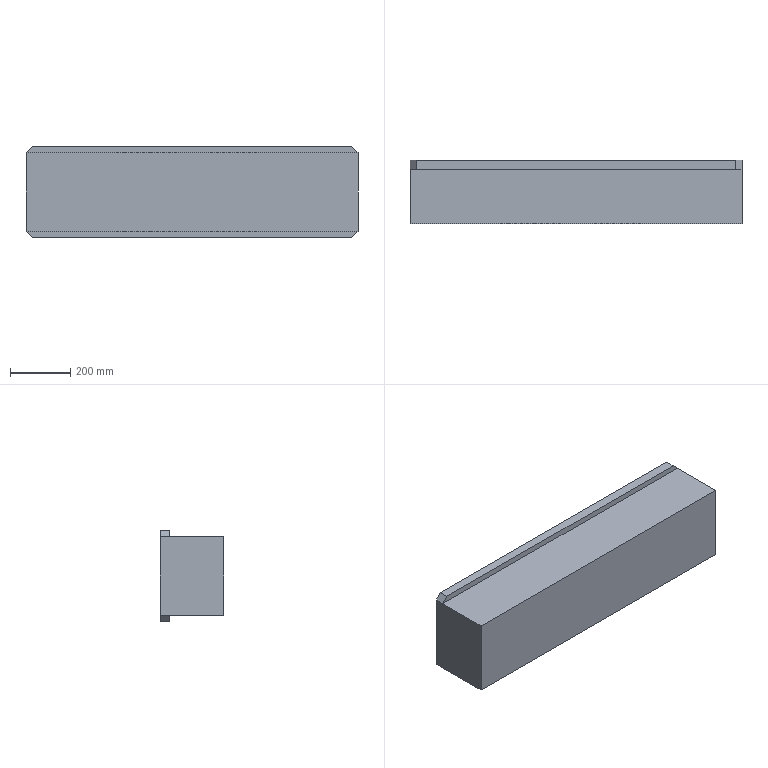Component | SolidWorks | -3[3]-1 | 1 solid | 26 faces | box 1100 x 210 x 300 mm | volume 61122548 mm3 | plane 18 | cylinder 8 | commonest cylinder face diameters 65 x4 27 x4
STEP:
#1=COLOUR_RGB('',0.7922,0.8196,0.9333);
#2=FILL_AREA_STYLE_COLOUR('',#1);
#3=FILL_AREA_STYLE('',(#2));
#4=SURFACE_STYLE_FILL_AREA(#3);
#5=SURFACE_SIDE_STYLE('',(#4));
#6=SURFACE_STYLE_USAGE(.BOTH.,#5);
#7=PRESENTATION_STYLE_ASSIGNMENT((#6));
#8=CARTESIAN_POINT('',(19.685,-89.764,47.736));
#9=VERTEX_POINT('',#8);
#10=CARTESIAN_POINT('',(19.685,-89.764,45.177));
#11=VERTEX_POINT('',#10);
#12=CARTESIAN_POINT('',(19.685,-89.764,46.457));
#13=DIRECTION('',(0.,-1.,0.));
#14=DIRECTION('',(0.,0.,1.));
#15=AXIS2_PLACEMENT_3D('',#12,#13,#14);
#16=CIRCLE('',#15,1.28);
#17=EDGE_CURVE('',#9,#11,#16,.T.);
#18=ORIENTED_EDGE('',*,*,#17,.T.);
#19=CARTESIAN_POINT('',(19.685,-88.583,45.177));
#20=VERTEX_POINT('',#19);
#21=CARTESIAN_POINT('',(19.685,-89.764,45.177));
#22=DIRECTION('',(0.,1.,0.));
#23=VECTOR('',#22,39.37);
#24=LINE('',#21,#23);
#25=EDGE_CURVE('',#11,#20,#24,.T.);
#26=ORIENTED_EDGE('',*,*,#25,.T.);
#27=CARTESIAN_POINT('',(19.685,-88.583,47.736));
#28=VERTEX_POINT('',#27);
#29=CARTESIAN_POINT('',(19.685,-88.583,46.457));
#30=DIRECTION('',(0.,-1.,0.));
#31=DIRECTION('',(0.,0.,1.));
#32=AXIS2_PLACEMENT_3D('',#29,#30,#31);
#33=CIRCLE('',#32,1.28);
#34=EDGE_CURVE('',#28,#20,#33,.T.);
#35=ORIENTED_EDGE('',*,*,#34,.F.);
#36=CARTESIAN_POINT('',(19.685,-89.764,47.736));
#37=DIRECTION('',(0.,1.,0.));
#38=VECTOR('',#37,39.37);
#39=LINE('',#36,#38);
#40=EDGE_CURVE('',#9,#28,#39,.T.);
#41=ORIENTED_EDGE('',*,*,#40,.F.);
#42=EDGE_LOOP('',(#18,#26,#35,#41));
#43=FACE_OUTER_BOUND('',#42,.T.);
#44=CARTESIAN_POINT('',(19.685,-89.764,46.457));
#45=DIRECTION('',(0.,1.,0.));
#46=DIRECTION('',(0.,0.,-1.));
#47=AXIS2_PLACEMENT_3D('',#44,#45,#46);
#48=CYLINDRICAL_SURFACE('',#47,1.28);
#49=ADVANCED_FACE('',(#43),#48,.F.);
#50=CARTESIAN_POINT('',(19.685,-89.764,43.839));
#51=VERTEX_POINT('',#50);
#52=CARTESIAN_POINT('',(19.685,-89.764,42.776));
#53=VERTEX_POINT('',#52);
#54=CARTESIAN_POINT('',(19.685,-89.764,43.307));
#55=DIRECTION('',(0.,-1.,0.));
#56=DIRECTION('',(0.,0.,1.));
#57=AXIS2_PLACEMENT_3D('',#54,#55,#56);
#58=CIRCLE('',#57,0.5315);
#59=EDGE_CURVE('',#51,#53,#58,.T.);
#60=ORIENTED_EDGE('',*,*,#59,.T.);
#61=CARTESIAN_POINT('',(19.685,-88.583,42.776));
#62=VERTEX_POINT('',#61);
#63=CARTESIAN_POINT('',(19.685,-89.764,42.776));
#64=DIRECTION('',(0.,1.,0.));
#65=VECTOR('',#64,39.37);
#66=LINE('',#63,#65);
#67=EDGE_CURVE('',#53,#62,#66,.T.);
#68=ORIENTED_EDGE('',*,*,#67,.T.);
#69=CARTESIAN_POINT('',(19.685,-88.583,43.839));
#70=VERTEX_POINT('',#69);
#71=CARTESIAN_POINT('',(19.685,-88.583,43.307));
#72=DIRECTION('',(0.,-1.,0.));
#73=DIRECTION('',(0.,0.,1.));
#74=AXIS2_PLACEMENT_3D('',#71,#72,#73);
#75=CIRCLE('',#74,0.5315);
#76=EDGE_CURVE('',#70,#62,#75,.T.);
#77=ORIENTED_EDGE('',*,*,#76,.F.);
#78=CARTESIAN_POINT('',(19.685,-89.764,43.839));
#79=DIRECTION('',(0.,1.,0.));
#80=VECTOR('',#79,39.37);
#81=LINE('',#78,#80);
#82=EDGE_CURVE('',#51,#70,#81,.T.);
#83=ORIENTED_EDGE('',*,*,#82,.F.);
#84=EDGE_LOOP('',(#60,#68,#77,#83));
#85=FACE_OUTER_BOUND('',#84,.T.);
#86=CARTESIAN_POINT('',(19.685,-89.764,43.307));
#87=DIRECTION('',(0.,1.,0.));
#88=DIRECTION('',(0.,0.,-1.));
#89=AXIS2_PLACEMENT_3D('',#86,#87,#88);
#90=CYLINDRICAL_SURFACE('',#89,0.5315);
#91=ADVANCED_FACE('',(#85),#90,.F.);
#92=CARTESIAN_POINT('',(-19.685,-89.764,43.839));
#93=VERTEX_POINT('',#92);
#94=CARTESIAN_POINT('',(-19.685,-89.764,42.776));
#95=VERTEX_POINT('',#94);
#96=CARTESIAN_POINT('',(-19.685,-89.764,43.307));
#97=DIRECTION('',(0.,-1.,0.));
#98=DIRECTION('',(0.,0.,-1.));
#99=AXIS2_PLACEMENT_3D('',#96,#97,#98);
#100=CIRCLE('',#99,0.5315);
#101=EDGE_CURVE('',#93,#95,#100,.T.);
#102=ORIENTED_EDGE('',*,*,#101,.T.);
#103=CARTESIAN_POINT('',(-19.685,-88.583,42.776));
#104=VERTEX_POINT('',#103);
#105=CARTESIAN_POINT('',(-19.685,-89.764,42.776));
#106=DIRECTION('',(0.,1.,0.));
#107=VECTOR('',#106,39.37);
#108=LINE('',#105,#107);
#109=EDGE_CURVE('',#95,#104,#108,.T.);
#110=ORIENTED_EDGE('',*,*,#109,.T.);
#111=CARTESIAN_POINT('',(-19.685,-88.583,43.839));
#112=VERTEX_POINT('',#111);
#113=CARTESIAN_POINT('',(-19.685,-88.583,43.307));
#114=DIRECTION('',(0.,-1.,0.));
#115=DIRECTION('',(0.,0.,-1.));
#116=AXIS2_PLACEMENT_3D('',#113,#114,#115);
#117=CIRCLE('',#116,0.5315);
#118=EDGE_CURVE('',#112,#104,#117,.T.);
#119=ORIENTED_EDGE('',*,*,#118,.F.);
#120=CARTESIAN_POINT('',(-19.685,-89.764,43.839));
#121=DIRECTION('',(0.,1.,0.));
#122=VECTOR('',#121,39.37);
#123=LINE('',#120,#122);
#124=EDGE_CURVE('',#93,#112,#123,.T.);
#125=ORIENTED_EDGE('',*,*,#124,.F.);
#126=EDGE_LOOP('',(#102,#110,#119,#125));
#127=FACE_OUTER_BOUND('',#126,.T.);
#128=CARTESIAN_POINT('',(-19.685,-89.764,43.307));
#129=DIRECTION('',(0.,1.,0.));
#130=DIRECTION('',(0.,0.,-1.));
#131=AXIS2_PLACEMENT_3D('',#128,#129,#130);
#132=CYLINDRICAL_SURFACE('',#131,0.5315);
#133=ADVANCED_FACE('',(#127),#132,.F.);
#134=CARTESIAN_POINT('',(-19.685,-89.764,47.736));
#135=VERTEX_POINT('',#134);
#136=CARTESIAN_POINT('',(-19.685,-89.764,45.177));
#137=VERTEX_POINT('',#136);
#138=CARTESIAN_POINT('',(-19.685,-89.764,46.457));
#139=DIRECTION('',(0.,-1.,0.));
#140=DIRECTION('',(0.,0.,-1.));
#141=AXIS2_PLACEMENT_3D('',#138,#139,#140);
#142=CIRCLE('',#141,1.28);
#143=EDGE_CURVE('',#135,#137,#142,.T.);
#144=ORIENTED_EDGE('',*,*,#143,.T.);
#145=CARTESIAN_POINT('',(-19.685,-88.583,45.177));
#146=VERTEX_POINT('',#145);
#147=CARTESIAN_POINT('',(-19.685,-89.764,45.177));
#148=DIRECTION('',(0.,1.,0.));
#149=VECTOR('',#148,39.37);
#150=LINE('',#147,#149);
#151=EDGE_CURVE('',#137,#146,#150,.T.);
#152=ORIENTED_EDGE('',*,*,#151,.T.);
#153=CARTESIAN_POINT('',(-19.685,-88.583,47.736));
#154=VERTEX_POINT('',#153);
#155=CARTESIAN_POINT('',(-19.685,-88.583,46.457));
#156=DIRECTION('',(0.,-1.,0.));
#157=DIRECTION('',(0.,0.,-1.));
#158=AXIS2_PLACEMENT_3D('',#155,#156,#157);
#159=CIRCLE('',#158,1.28);
#160=EDGE_CURVE('',#154,#146,#159,.T.);
#161=ORIENTED_EDGE('',*,*,#160,.F.);
#162=CARTESIAN_POINT('',(-19.685,-89.764,47.736));
#163=DIRECTION('',(0.,1.,0.));
#164=VECTOR('',#163,39.37);
#165=LINE('',#162,#164);
#166=EDGE_CURVE('',#135,#154,#165,.T.);
#167=ORIENTED_EDGE('',*,*,#166,.F.);
#168=EDGE_LOOP('',(#144,#152,#161,#167));
#169=FACE_OUTER_BOUND('',#168,.T.);
#170=CARTESIAN_POINT('',(-19.685,-89.764,46.457));
#171=DIRECTION('',(0.,1.,0.));
#172=DIRECTION('',(0.,0.,-1.));
#173=AXIS2_PLACEMENT_3D('',#170,#171,#172);
#174=CYLINDRICAL_SURFACE('',#173,1.28);
#175=ADVANCED_FACE('',(#169),#174,.F.);
#176=CARTESIAN_POINT('',(21.654,-89.764,50.394));
#177=VERTEX_POINT('',#176);
#178=CARTESIAN_POINT('',(-21.654,-89.764,50.394));
#179=VERTEX_POINT('',#178);
#180=CARTESIAN_POINT('',(-21.654,-89.764,50.394));
#181=DIRECTION('',(-1.,0.,0.));
#182=VECTOR('',#181,39.37);
#183=LINE('',#180,#182);
#184=EDGE_CURVE('',#177,#179,#183,.T.);
#185=ORIENTED_EDGE('',*,*,#184,.F.);
#186=CARTESIAN_POINT('',(20.866,-89.764,51.181));
#187=VERTEX_POINT('',#186);
#188=CARTESIAN_POINT('',(20.866,-89.764,51.181));
#189=DIRECTION('',(-0.7071,0.,0.7071));
#190=VECTOR('',#189,39.37);
#191=LINE('',#188,#190);
#192=EDGE_CURVE('',#177,#187,#191,.T.);
#193=ORIENTED_EDGE('',*,*,#192,.T.);
#194=CARTESIAN_POINT('',(-20.866,-89.764,51.181));
#195=VERTEX_POINT('',#194);
#196=CARTESIAN_POINT('',(-20.866,-89.764,51.181));
#197=DIRECTION('',(-1.,0.,-0.));
#198=VECTOR('',#197,39.37);
#199=LINE('',#196,#198);
#200=EDGE_CURVE('',#187,#195,#199,.T.);
#201=ORIENTED_EDGE('',*,*,#200,.T.);
#202=CARTESIAN_POINT('',(-21.654,-89.764,50.394));
#203=DIRECTION('',(-0.7071,0.,-0.7071));
#204=VECTOR('',#203,39.37);
#205=LINE('',#202,#204);
#206=EDGE_CURVE('',#195,#179,#205,.T.);
#207=ORIENTED_EDGE('',*,*,#206,.T.);
#208=EDGE_LOOP('',(#185,#193,#201,#207));
#209=FACE_OUTER_BOUND('',#208,.T.);
#210=CARTESIAN_POINT('',(0.,-89.764,72.047));
#211=DIRECTION('',(0.,1.,0.));
#212=DIRECTION('',(0.,0.,-1.));
#213=AXIS2_PLACEMENT_3D('',#210,#211,#212);
#214=PLANE('',#213);
#215=ADVANCED_FACE('',(#209),#214,.F.);
#216=CARTESIAN_POINT('',(-21.654,-89.764,40.157));
#217=VERTEX_POINT('',#216);
#218=CARTESIAN_POINT('',(21.654,-89.764,40.157));
#219=VERTEX_POINT('',#218);
#220=CARTESIAN_POINT('',(-21.654,-89.764,40.157));
#221=DIRECTION('',(1.,0.,0.));
#222=VECTOR('',#221,39.37);
#223=LINE('',#220,#222);
#224=EDGE_CURVE('',#217,#219,#223,.T.);
#225=ORIENTED_EDGE('',*,*,#224,.F.);
#226=CARTESIAN_POINT('',(-20.866,-89.764,39.37));
#227=VERTEX_POINT('',#226);
#228=CARTESIAN_POINT('',(-21.654,-89.764,40.157));
#229=DIRECTION('',(0.7071,0.,-0.7071));
#230=VECTOR('',#229,39.37);
#231=LINE('',#228,#230);
#232=EDGE_CURVE('',#217,#227,#231,.T.);
#233=ORIENTED_EDGE('',*,*,#232,.T.);
#234=CARTESIAN_POINT('',(20.866,-89.764,39.37));
#235=VERTEX_POINT('',#234);
#236=CARTESIAN_POINT('',(-20.866,-89.764,39.37));
#237=DIRECTION('',(1.,0.,0.));
#238=VECTOR('',#237,39.37);
#239=LINE('',#236,#238);
#240=EDGE_CURVE('',#227,#235,#239,.T.);
#241=ORIENTED_EDGE('',*,*,#240,.T.);
#242=CARTESIAN_POINT('',(21.654,-89.764,40.157));
#243=DIRECTION('',(0.7071,0.,0.7071));
#244=VECTOR('',#243,39.37);
#245=LINE('',#242,#244);
#246=EDGE_CURVE('',#235,#219,#245,.T.);
#247=ORIENTED_EDGE('',*,*,#246,.T.);
#248=EDGE_LOOP('',(#225,#233,#241,#247));
#249=FACE_OUTER_BOUND('',#248,.T.);
#250=CARTESIAN_POINT('',(0.,-89.764,72.047));
#251=DIRECTION('',(0.,1.,0.));
#252=DIRECTION('',(0.,0.,-1.));
#253=AXIS2_PLACEMENT_3D('',#250,#251,#252);
#254=PLANE('',#253);
#255=ADVANCED_FACE('',(#249),#254,.F.);
#256=ORIENTED_EDGE('',*,*,#76,.T.);
#257=CARTESIAN_POINT('',(19.685,-88.583,43.307));
#258=DIRECTION('',(0.,-1.,0.));
#259=DIRECTION('',(0.,0.,1.));
#260=AXIS2_PLACEMENT_3D('',#257,#258,#259);
#261=CIRCLE('',#260,0.5315);
#262=EDGE_CURVE('',#62,#70,#261,.T.);
#263=ORIENTED_EDGE('',*,*,#262,.T.);
#264=EDGE_LOOP('',(#256,#263));
#265=FACE_BOUND('',#264,.T.);
#266=ORIENTED_EDGE('',*,*,#160,.T.);
#267=CARTESIAN_POINT('',(-19.685,-88.583,46.457));
#268=DIRECTION('',(0.,-1.,0.));
#269=DIRECTION('',(0.,0.,-1.));
#270=AXIS2_PLACEMENT_3D('',#267,#268,#269);
#271=CIRCLE('',#270,1.28);
#272=EDGE_CURVE('',#146,#154,#271,.T.);
#273=ORIENTED_EDGE('',*,*,#272,.T.);
#274=EDGE_LOOP('',(#266,#273));
#275=FACE_BOUND('',#274,.T.);
#276=CARTESIAN_POINT('',(-20.866,-88.583,51.181));
#277=VERTEX_POINT('',#276);
#278=CARTESIAN_POINT('',(-21.654,-88.583,50.394));
#279=VERTEX_POINT('',#278);
#280=CARTESIAN_POINT('',(-21.654,-88.583,50.394));
#281=DIRECTION('',(-0.7071,0.,-0.7071));
#282=VECTOR('',#281,39.37);
#283=LINE('',#280,#282);
#284=EDGE_CURVE('',#277,#279,#283,.T.);
#285=ORIENTED_EDGE('',*,*,#284,.F.);
#286=CARTESIAN_POINT('',(20.866,-88.583,51.181));
#287=VERTEX_POINT('',#286);
#288=CARTESIAN_POINT('',(-20.866,-88.583,51.181));
#289=DIRECTION('',(-1.,0.,-0.));
#290=VECTOR('',#289,39.37);
#291=LINE('',#288,#290);
#292=EDGE_CURVE('',#287,#277,#291,.T.);
#293=ORIENTED_EDGE('',*,*,#292,.F.);
#294=CARTESIAN_POINT('',(21.654,-88.583,50.394));
#295=VERTEX_POINT('',#294);
#296=CARTESIAN_POINT('',(20.866,-88.583,51.181));
#297=DIRECTION('',(-0.7071,0.,0.7071));
#298=VECTOR('',#297,39.37);
#299=LINE('',#296,#298);
#300=EDGE_CURVE('',#295,#287,#299,.T.);
#301=ORIENTED_EDGE('',*,*,#300,.F.);
#302=CARTESIAN_POINT('',(21.654,-88.583,40.157));
#303=VERTEX_POINT('',#302);
#304=CARTESIAN_POINT('',(21.654,-88.583,50.394));
#305=DIRECTION('',(0.,0.,1.));
#306=VECTOR('',#305,39.37);
#307=LINE('',#304,#306);
#308=EDGE_CURVE('',#303,#295,#307,.T.);
#309=ORIENTED_EDGE('',*,*,#308,.F.);
#310=CARTESIAN_POINT('',(20.866,-88.583,39.37));
#311=VERTEX_POINT('',#310);
#312=CARTESIAN_POINT('',(21.654,-88.583,40.157));
#313=DIRECTION('',(0.7071,0.,0.7071));
#314=VECTOR('',#313,39.37);
#315=LINE('',#312,#314);
#316=EDGE_CURVE('',#311,#303,#315,.T.);
#317=ORIENTED_EDGE('',*,*,#316,.F.);
#318=CARTESIAN_POINT('',(-20.866,-88.583,39.37));
#319=VERTEX_POINT('',#318);
#320=CARTESIAN_POINT('',(-20.866,-88.583,39.37));
#321=DIRECTION('',(1.,0.,0.));
#322=VECTOR('',#321,39.37);
#323=LINE('',#320,#322);
#324=EDGE_CURVE('',#319,#311,#323,.T.);
#325=ORIENTED_EDGE('',*,*,#324,.F.);
#326=CARTESIAN_POINT('',(-21.654,-88.583,40.157));
#327=VERTEX_POINT('',#326);
#328=CARTESIAN_POINT('',(-21.654,-88.583,40.157));
#329=DIRECTION('',(0.7071,0.,-0.7071));
#330=VECTOR('',#329,39.37);
#331=LINE('',#328,#330);
#332=EDGE_CURVE('',#327,#319,#331,.T.);
#333=ORIENTED_EDGE('',*,*,#332,.F.);
#334=CARTESIAN_POINT('',(-21.654,-88.583,50.394));
#335=DIRECTION('',(0.,0.,-1.));
#336=VECTOR('',#335,39.37);
#337=LINE('',#334,#336);
#338=EDGE_CURVE('',#279,#327,#337,.T.);
#339=ORIENTED_EDGE('',*,*,#338,.F.);
#340=EDGE_LOOP('',(#285,#293,#301,#309,#317,#325,#333,#339));
#341=FACE_OUTER_BOUND('',#340,.T.);
#342=ORIENTED_EDGE('',*,*,#118,.T.);
#343=CARTESIAN_POINT('',(-19.685,-88.583,43.307));
#344=DIRECTION('',(0.,-1.,0.));
#345=DIRECTION('',(0.,0.,-1.));
#346=AXIS2_PLACEMENT_3D('',#343,#344,#345);
#347=CIRCLE('',#346,0.5315);
#348=EDGE_CURVE('',#104,#112,#347,.T.);
#349=ORIENTED_EDGE('',*,*,#348,.T.);
#350=EDGE_LOOP('',(#342,#349));
#351=FACE_BOUND('',#350,.T.);
#352=ORIENTED_EDGE('',*,*,#34,.T.);
#353=CARTESIAN_POINT('',(19.685,-88.583,46.457));
#354=DIRECTION('',(0.,-1.,0.));
#355=DIRECTION('',(0.,0.,1.));
#356=AXIS2_PLACEMENT_3D('',#353,#354,#355);
#357=CIRCLE('',#356,1.28);
#358=EDGE_CURVE('',#20,#28,#357,.T.);
#359=ORIENTED_EDGE('',*,*,#358,.T.);
#360=EDGE_LOOP('',(#352,#359));
#361=FACE_BOUND('',#360,.T.);
#362=CARTESIAN_POINT('',(0.,-88.583,72.047));
#363=DIRECTION('',(0.,1.,0.));
#364=DIRECTION('',(0.,0.,-1.));
#365=AXIS2_PLACEMENT_3D('',#362,#363,#364);
#366=PLANE('',#365);
#367=ADVANCED_FACE('',(#265,#275,#341,#351,#361),#366,.T.);
#368=ORIENTED_EDGE('',*,*,#284,.T.);
#369=CARTESIAN_POINT('',(-21.654,-89.764,50.394));
#370=DIRECTION('',(0.,1.,0.));
#371=VECTOR('',#370,39.37);
#372=LINE('',#369,#371);
#373=EDGE_CURVE('',#179,#279,#372,.T.);
#374=ORIENTED_EDGE('',*,*,#373,.F.);
#375=ORIENTED_EDGE('',*,*,#206,.F.);
#376=CARTESIAN_POINT('',(-20.866,-89.764,51.181));
#377=DIRECTION('',(0.,1.,0.));
#378=VECTOR('',#377,39.37);
#379=LINE('',#376,#378);
#380=EDGE_CURVE('',#195,#277,#379,.T.);
#381=ORIENTED_EDGE('',*,*,#380,.T.);
#382=EDGE_LOOP('',(#368,#374,#375,#381));
#383=FACE_OUTER_BOUND('',#382,.T.);
#384=CARTESIAN_POINT('',(-21.654,-89.764,50.394));
#385=DIRECTION('',(0.7071,0.,-0.7071));
#386=DIRECTION('',(0.7071,0.,0.7071));
#387=AXIS2_PLACEMENT_3D('',#384,#385,#386);
#388=PLANE('',#387);
#389=ADVANCED_FACE('',(#383),#388,.F.);
#390=ORIENTED_EDGE('',*,*,#338,.T.);
#391=CARTESIAN_POINT('',(-21.654,-89.764,40.157));
#392=DIRECTION('',(0.,1.,0.));
#393=VECTOR('',#392,39.37);
#394=LINE('',#391,#393);
#395=EDGE_CURVE('',#217,#327,#394,.T.);
#396=ORIENTED_EDGE('',*,*,#395,.F.);
#397=CARTESIAN_POINT('',(-21.654,-96.85,40.157));
#398=VERTEX_POINT('',#397);
#399=CARTESIAN_POINT('',(-21.654,-96.85,40.157));
#400=DIRECTION('',(0.,1.,0.));
#401=VECTOR('',#400,39.37);
#402=LINE('',#399,#401);
#403=EDGE_CURVE('',#398,#217,#402,.T.);
#404=ORIENTED_EDGE('',*,*,#403,.F.);
#405=CARTESIAN_POINT('',(-21.654,-96.85,50.394));
#406=VERTEX_POINT('',#405);
#407=CARTESIAN_POINT('',(-21.654,-96.85,50.394));
#408=DIRECTION('',(0.,0.,-1.));
#409=VECTOR('',#408,39.37);
#410=LINE('',#407,#409);
#411=EDGE_CURVE('',#406,#398,#410,.T.);
#412=ORIENTED_EDGE('',*,*,#411,.F.);
#413=CARTESIAN_POINT('',(-21.654,-96.85,50.394));
#414=DIRECTION('',(0.,1.,0.));
#415=VECTOR('',#414,39.37);
#416=LINE('',#413,#415);
#417=EDGE_CURVE('',#406,#179,#416,.T.);
#418=ORIENTED_EDGE('',*,*,#417,.T.);
#419=ORIENTED_EDGE('',*,*,#373,.T.);
#420=EDGE_LOOP('',(#390,#396,#404,#412,#418,#419));
#421=FACE_OUTER_BOUND('',#420,.T.);
#422=CARTESIAN_POINT('',(-21.654,-89.764,50.394));
#423=DIRECTION('',(1.,0.,0.));
#424=DIRECTION('',(-0.,0.,1.));
#425=AXIS2_PLACEMENT_3D('',#422,#423,#424);
#426=PLANE('',#425);
#427=ADVANCED_FACE('',(#421),#426,.F.);
#428=ORIENTED_EDGE('',*,*,#332,.T.);
#429=CARTESIAN_POINT('',(-20.866,-89.764,39.37));
#430=DIRECTION('',(0.,1.,0.));
#431=VECTOR('',#430,39.37);
#432=LINE('',#429,#431);
#433=EDGE_CURVE('',#227,#319,#432,.T.);
#434=ORIENTED_EDGE('',*,*,#433,.F.);
#435=ORIENTED_EDGE('',*,*,#232,.F.);
#436=ORIENTED_EDGE('',*,*,#395,.T.);
#437=EDGE_LOOP('',(#428,#434,#435,#436));
#438=FACE_OUTER_BOUND('',#437,.T.);
#439=CARTESIAN_POINT('',(-21.654,-89.764,40.157));
#440=DIRECTION('',(0.7071,0.,0.7071));
#441=DIRECTION('',(-0.7071,0.,0.7071));
#442=AXIS2_PLACEMENT_3D('',#439,#440,#441);
#443=PLANE('',#442);
#444=ADVANCED_FACE('',(#438),#443,.F.);
#445=ORIENTED_EDGE('',*,*,#324,.T.);
#446=CARTESIAN_POINT('',(20.866,-89.764,39.37));
#447=DIRECTION('',(0.,1.,0.));
#448=VECTOR('',#447,39.37);
#449=LINE('',#446,#448);
#450=EDGE_CURVE('',#235,#311,#449,.T.);
#451=ORIENTED_EDGE('',*,*,#450,.F.);
#452=ORIENTED_EDGE('',*,*,#240,.F.);
#453=ORIENTED_EDGE('',*,*,#433,.T.);
#454=EDGE_LOOP('',(#445,#451,#452,#453));
#455=FACE_OUTER_BOUND('',#454,.T.);
#456=CARTESIAN_POINT('',(-20.866,-89.764,39.37));
#457=DIRECTION('',(-0.,0.,1.));
#458=DIRECTION('',(-1.,0.,-0.));
#459=AXIS2_PLACEMENT_3D('',#456,#457,#458);
#460=PLANE('',#459);
#461=ADVANCED_FACE('',(#455),#460,.F.);
#462=ORIENTED_EDGE('',*,*,#316,.T.);
#463=CARTESIAN_POINT('',(21.654,-89.764,40.157));
#464=DIRECTION('',(0.,1.,0.));
#465=VECTOR('',#464,39.37);
#466=LINE('',#463,#465);
#467=EDGE_CURVE('',#219,#303,#466,.T.);
#468=ORIENTED_EDGE('',*,*,#467,.F.);
#469=ORIENTED_EDGE('',*,*,#246,.F.);
#470=ORIENTED_EDGE('',*,*,#450,.T.);
#471=EDGE_LOOP('',(#462,#468,#469,#470));
#472=FACE_OUTER_BOUND('',#471,.T.);
#473=CARTESIAN_POINT('',(21.654,-89.764,40.157));
#474=DIRECTION('',(-0.7071,0.,0.7071));
#475=DIRECTION('',(-0.7071,0.,-0.7071));
#476=AXIS2_PLACEMENT_3D('',#473,#474,#475);
#477=PLANE('',#476);
#478=ADVANCED_FACE('',(#472),#477,.F.);
#479=ORIENTED_EDGE('',*,*,#308,.T.);
#480=CARTESIAN_POINT('',(21.654,-89.764,50.394));
#481=DIRECTION('',(0.,1.,0.));
#482=VECTOR('',#481,39.37);
#483=LINE('',#480,#482);
#484=EDGE_CURVE('',#177,#295,#483,.T.);
#485=ORIENTED_EDGE('',*,*,#484,.F.);
#486=CARTESIAN_POINT('',(21.654,-96.85,50.394));
#487=VERTEX_POINT('',#486);
#488=CARTESIAN_POINT('',(21.654,-96.85,50.394));
#489=DIRECTION('',(0.,1.,0.));
#490=VECTOR('',#489,39.37);
#491=LINE('',#488,#490);
#492=EDGE_CURVE('',#487,#177,#491,.T.);
#493=ORIENTED_EDGE('',*,*,#492,.F.);
#494=CARTESIAN_POINT('',(21.654,-96.85,40.157));
#495=VERTEX_POINT('',#494);
#496=CARTESIAN_POINT('',(21.654,-96.85,50.394));
#497=DIRECTION('',(0.,0.,1.));
#498=VECTOR('',#497,39.37);
#499=LINE('',#496,#498);
#500=EDGE_CURVE('',#495,#487,#499,.T.);
#501=ORIENTED_EDGE('',*,*,#500,.F.);
#502=CARTESIAN_POINT('',(21.654,-96.85,40.157));
#503=DIRECTION('',(0.,1.,0.));
#504=VECTOR('',#503,39.37);
#505=LINE('',#502,#504);
#506=EDGE_CURVE('',#495,#219,#505,.T.);
#507=ORIENTED_EDGE('',*,*,#506,.T.);
#508=ORIENTED_EDGE('',*,*,#467,.T.);
#509=EDGE_LOOP('',(#479,#485,#493,#501,#507,#508));
#510=FACE_OUTER_BOUND('',#509,.T.);
#511=CARTESIAN_POINT('',(21.654,-89.764,50.394));
#512=DIRECTION('',(-1.,0.,0.));
#513=DIRECTION('',(-0.,0.,-1.));
#514=AXIS2_PLACEMENT_3D('',#511,#512,#513);
#515=PLANE('',#514);
#516=ADVANCED_FACE('',(#510),#515,.F.);
#517=ORIENTED_EDGE('',*,*,#300,.T.);
#518=CARTESIAN_POINT('',(20.866,-89.764,51.181));
#519=DIRECTION('',(0.,1.,0.));
#520=VECTOR('',#519,39.37);
#521=LINE('',#518,#520);
#522=EDGE_CURVE('',#187,#287,#521,.T.);
#523=ORIENTED_EDGE('',*,*,#522,.F.);
#524=ORIENTED_EDGE('',*,*,#192,.F.);
#525=ORIENTED_EDGE('',*,*,#484,.T.);
#526=EDGE_LOOP('',(#517,#523,#524,#525));
#527=FACE_OUTER_BOUND('',#526,.T.);
#528=CARTESIAN_POINT('',(20.866,-89.764,51.181));
#529=DIRECTION('',(-0.7071,0.,-0.7071));
#530=DIRECTION('',(0.7071,0.,-0.7071));
#531=AXIS2_PLACEMENT_3D('',#528,#529,#530);
#532=PLANE('',#531);
#533=ADVANCED_FACE('',(#527),#532,.F.);
#534=ORIENTED_EDGE('',*,*,#292,.T.);
#535=ORIENTED_EDGE('',*,*,#380,.F.);
#536=ORIENTED_EDGE('',*,*,#200,.F.);
#537=ORIENTED_EDGE('',*,*,#522,.T.);
#538=EDGE_LOOP('',(#534,#535,#536,#537));
#539=FACE_OUTER_BOUND('',#538,.T.);
#540=CARTESIAN_POINT('',(-20.866,-89.764,51.181));
#541=DIRECTION('',(0.,0.,-1.));
#542=DIRECTION('',(1.,0.,0.));
#543=AXIS2_PLACEMENT_3D('',#540,#541,#542);
#544=PLANE('',#543);
#545=ADVANCED_FACE('',(#539),#544,.F.);
#546=ORIENTED_EDGE('',*,*,#151,.F.);
#547=CARTESIAN_POINT('',(-19.685,-89.764,46.457));
#548=DIRECTION('',(0.,-1.,0.));
#549=DIRECTION('',(0.,0.,-1.));
#550=AXIS2_PLACEMENT_3D('',#547,#548,#549);
#551=CIRCLE('',#550,1.28);
#552=EDGE_CURVE('',#137,#135,#551,.T.);
#553=ORIENTED_EDGE('',*,*,#552,.T.);
#554=ORIENTED_EDGE('',*,*,#166,.T.);
#555=ORIENTED_EDGE('',*,*,#272,.F.);
#556=EDGE_LOOP('',(#546,#553,#554,#555));
#557=FACE_OUTER_BOUND('',#556,.T.);
#558=CARTESIAN_POINT('',(-19.685,-89.764,46.457));
#559=DIRECTION('',(0.,1.,0.));
#560=DIRECTION('',(0.,0.,-1.));
#561=AXIS2_PLACEMENT_3D('',#558,#559,#560);
#562=CYLINDRICAL_SURFACE('',#561,1.28);
#563=ADVANCED_FACE('',(#557),#562,.F.);
#564=ORIENTED_EDGE('',*,*,#109,.F.);
#565=CARTESIAN_POINT('',(-19.685,-89.764,43.307));
#566=DIRECTION('',(0.,-1.,0.));
#567=DIRECTION('',(0.,0.,-1.));
#568=AXIS2_PLACEMENT_3D('',#565,#566,#567);
#569=CIRCLE('',#568,0.5315);
#570=EDGE_CURVE('',#95,#93,#569,.T.);
#571=ORIENTED_EDGE('',*,*,#570,.T.);
#572=ORIENTED_EDGE('',*,*,#124,.T.);
#573=ORIENTED_EDGE('',*,*,#348,.F.);
#574=EDGE_LOOP('',(#564,#571,#572,#573));
#575=FACE_OUTER_BOUND('',#574,.T.);
#576=CARTESIAN_POINT('',(-19.685,-89.764,43.307));
#577=DIRECTION('',(0.,1.,0.));
#578=DIRECTION('',(0.,0.,-1.));
#579=AXIS2_PLACEMENT_3D('',#576,#577,#578);
#580=CYLINDRICAL_SURFACE('',#579,0.5315);
#581=ADVANCED_FACE('',(#575),#580,.F.);
#582=ORIENTED_EDGE('',*,*,#67,.F.);
#583=CARTESIAN_POINT('',(19.685,-89.764,43.307));
#584=DIRECTION('',(0.,-1.,0.));
#585=DIRECTION('',(0.,0.,1.));
#586=AXIS2_PLACEMENT_3D('',#583,#584,#585);
#587=CIRCLE('',#586,0.5315);
#588=EDGE_CURVE('',#53,#51,#587,.T.);
#589=ORIENTED_EDGE('',*,*,#588,.T.);
#590=ORIENTED_EDGE('',*,*,#82,.T.);
#591=ORIENTED_EDGE('',*,*,#262,.F.);
#592=EDGE_LOOP('',(#582,#589,#590,#591));
#593=FACE_OUTER_BOUND('',#592,.T.);
#594=CARTESIAN_POINT('',(19.685,-89.764,43.307));
#595=DIRECTION('',(0.,1.,0.));
#596=DIRECTION('',(0.,0.,-1.));
#597=AXIS2_PLACEMENT_3D('',#594,#595,#596);
#598=CYLINDRICAL_SURFACE('',#597,0.5315);
#599=ADVANCED_FACE('',(#593),#598,.F.);
#600=ORIENTED_EDGE('',*,*,#25,.F.);
#601=CARTESIAN_POINT('',(19.685,-89.764,46.457));
#602=DIRECTION('',(0.,-1.,0.));
#603=DIRECTION('',(0.,0.,1.));
#604=AXIS2_PLACEMENT_3D('',#601,#602,#603);
#605=CIRCLE('',#604,1.28);
#606=EDGE_CURVE('',#11,#9,#605,.T.);
#607=ORIENTED_EDGE('',*,*,#606,.T.);
#608=ORIENTED_EDGE('',*,*,#40,.T.);
#609=ORIENTED_EDGE('',*,*,#358,.F.);
#610=EDGE_LOOP('',(#600,#607,#608,#609));
#611=FACE_OUTER_BOUND('',#610,.T.);
#612=CARTESIAN_POINT('',(19.685,-89.764,46.457));
#613=DIRECTION('',(0.,1.,0.));
#614=DIRECTION('',(0.,0.,-1.));
#615=AXIS2_PLACEMENT_3D('',#612,#613,#614);
#616=CYLINDRICAL_SURFACE('',#615,1.28);
#617=ADVANCED_FACE('',(#611),#616,.F.);
#618=ORIENTED_EDGE('',*,*,#411,.T.);
#619=CARTESIAN_POINT('',(-21.654,-96.85,40.157));
#620=DIRECTION('',(1.,0.,0.));
#621=VECTOR('',#620,39.37);
#622=LINE('',#619,#621);
#623=EDGE_CURVE('',#398,#495,#622,.T.);
#624=ORIENTED_EDGE('',*,*,#623,.T.);
#625=ORIENTED_EDGE('',*,*,#500,.T.);
#626=CARTESIAN_POINT('',(-21.654,-96.85,50.394));
#627=DIRECTION('',(-1.,0.,0.));
#628=VECTOR('',#627,39.37);
#629=LINE('',#626,#628);
#630=EDGE_CURVE('',#487,#406,#629,.T.);
#631=ORIENTED_EDGE('',*,*,#630,.T.);
#632=EDGE_LOOP('',(#618,#624,#625,#631));
#633=FACE_OUTER_BOUND('',#632,.T.);
#634=CARTESIAN_POINT('',(0.,-96.85,0.));
#635=DIRECTION('',(0.,-1.,0.));
#636=DIRECTION('',(0.,0.,1.));
#637=AXIS2_PLACEMENT_3D('',#634,#635,#636);
#638=PLANE('',#637);
#639=ADVANCED_FACE('',(#633),#638,.T.);
#640=ORIENTED_EDGE('',*,*,#184,.T.);
#641=ORIENTED_EDGE('',*,*,#417,.F.);
#642=ORIENTED_EDGE('',*,*,#630,.F.);
#643=ORIENTED_EDGE('',*,*,#492,.T.);
#644=EDGE_LOOP('',(#640,#641,#642,#643));
#645=FACE_OUTER_BOUND('',#644,.T.);
#646=CARTESIAN_POINT('',(-21.654,-96.85,50.394));
#647=DIRECTION('',(0.,0.,-1.));
#648=DIRECTION('',(1.,0.,0.));
#649=AXIS2_PLACEMENT_3D('',#646,#647,#648);
#650=PLANE('',#649);
#651=ADVANCED_FACE('',(#645),#650,.F.);
#652=ORIENTED_EDGE('',*,*,#224,.T.);
#653=ORIENTED_EDGE('',*,*,#506,.F.);
#654=ORIENTED_EDGE('',*,*,#623,.F.);
#655=ORIENTED_EDGE('',*,*,#403,.T.);
#656=EDGE_LOOP('',(#652,#653,#654,#655));
#657=FACE_OUTER_BOUND('',#656,.T.);
#658=CARTESIAN_POINT('',(-21.654,-96.85,40.157));
#659=DIRECTION('',(0.,0.,1.));
#660=DIRECTION('',(-1.,0.,0.));
#661=AXIS2_PLACEMENT_3D('',#658,#659,#660);
#662=PLANE('',#661);
#663=ADVANCED_FACE('',(#657),#662,.F.);
#664=ORIENTED_EDGE('',*,*,#17,.F.);
#665=ORIENTED_EDGE('',*,*,#606,.F.);
#666=EDGE_LOOP('',(#664,#665));
#667=FACE_OUTER_BOUND('',#666,.T.);
#668=CARTESIAN_POINT('',(0.,-89.764,0.));
#669=DIRECTION('',(0.,-1.,0.));
#670=DIRECTION('',(0.,0.,1.));
#671=AXIS2_PLACEMENT_3D('',#668,#669,#670);
#672=PLANE('',#671);
#673=ADVANCED_FACE('',(#667),#672,.F.);
#674=ORIENTED_EDGE('',*,*,#101,.F.);
#675=ORIENTED_EDGE('',*,*,#570,.F.);
#676=EDGE_LOOP('',(#674,#675));
#677=FACE_OUTER_BOUND('',#676,.T.);
#678=CARTESIAN_POINT('',(0.,-89.764,0.));
#679=DIRECTION('',(0.,-1.,0.));
#680=DIRECTION('',(0.,0.,1.));
#681=AXIS2_PLACEMENT_3D('',#678,#679,#680);
#682=PLANE('',#681);
#683=ADVANCED_FACE('',(#677),#682,.F.);
#684=ORIENTED_EDGE('',*,*,#143,.F.);
#685=ORIENTED_EDGE('',*,*,#552,.F.);
#686=EDGE_LOOP('',(#684,#685));
#687=FACE_OUTER_BOUND('',#686,.T.);
#688=CARTESIAN_POINT('',(0.,-89.764,0.));
#689=DIRECTION('',(0.,-1.,0.));
#690=DIRECTION('',(0.,0.,1.));
#691=AXIS2_PLACEMENT_3D('',#688,#689,#690);
#692=PLANE('',#691);
#693=ADVANCED_FACE('',(#687),#692,.F.);
#694=ORIENTED_EDGE('',*,*,#59,.F.);
#695=ORIENTED_EDGE('',*,*,#588,.F.);
#696=EDGE_LOOP('',(#694,#695));
#697=FACE_OUTER_BOUND('',#696,.T.);
#698=CARTESIAN_POINT('',(0.,-89.764,0.));
#699=DIRECTION('',(0.,-1.,0.));
#700=DIRECTION('',(0.,0.,1.));
#701=AXIS2_PLACEMENT_3D('',#698,#699,#700);
#702=PLANE('',#701);
#703=ADVANCED_FACE('',(#697),#702,.F.);
#704=CLOSED_SHELL('',(#49,#91,#133,#175,#215,#255,#367,#389,#427,#444,#461,#478,#516,#533,#545,#563,#581,#599,#617,#639,#651,#663,#673,#683,#693,#703));
#705=MANIFOLD_SOLID_BREP('',#704);
#706=STYLED_ITEM('',(#7),#705);
#707=(LENGTH_UNIT()NAMED_UNIT(*)SI_UNIT($,.METRE.));
#708=LENGTH_MEASURE_WITH_UNIT(LENGTH_MEASURE(0.0254),#707);
#709=DIMENSIONAL_EXPONENTS(1.,0.,0.,0.,0.,0.,0.);
#710=(CONVERSION_BASED_UNIT('',#708)LENGTH_UNIT()NAMED_UNIT(#709));
#711=UNCERTAINTY_MEASURE_WITH_UNIT(LENGTH_MEASURE(0.00001),#710,'','');
#712=(NAMED_UNIT(*)PLANE_ANGLE_UNIT()SI_UNIT($,.RADIAN.));
#713=(NAMED_UNIT(*)SI_UNIT($,.STERADIAN.)SOLID_ANGLE_UNIT());
#714=(GEOMETRIC_REPRESENTATION_CONTEXT(3)GLOBAL_UNCERTAINTY_ASSIGNED_CONTEXT((#711))GLOBAL_UNIT_ASSIGNED_CONTEXT((#710,#712,#713))REPRESENTATION_CONTEXT('',''));
#715=MECHANICAL_DESIGN_GEOMETRIC_PRESENTATION_REPRESENTATION('',(#706),#714);
#716=PRESENTATION_LAYER_ASSIGNMENT('','',(#706));
#717=CARTESIAN_POINT('',(0.,0.,0.));
#718=DIRECTION('',(0.,0.,1.));
#719=DIRECTION('',(1.,0.,0.));
#720=AXIS2_PLACEMENT_3D('',#717,#718,#719);
#721=(LENGTH_UNIT()NAMED_UNIT(*)SI_UNIT($,.METRE.));
#722=LENGTH_MEASURE_WITH_UNIT(LENGTH_MEASURE(0.0254),#721);
#723=DIMENSIONAL_EXPONENTS(1.,0.,0.,0.,0.,0.,0.);
#724=(CONVERSION_BASED_UNIT('',#722)LENGTH_UNIT()NAMED_UNIT(#723));
#725=UNCERTAINTY_MEASURE_WITH_UNIT(LENGTH_MEASURE(0.00001),#724,'','');
#726=(NAMED_UNIT(*)PLANE_ANGLE_UNIT()SI_UNIT($,.RADIAN.));
#727=(NAMED_UNIT(*)SI_UNIT($,.STERADIAN.)SOLID_ANGLE_UNIT());
#728=(GEOMETRIC_REPRESENTATION_CONTEXT(3)GLOBAL_UNCERTAINTY_ASSIGNED_CONTEXT((#725))GLOBAL_UNIT_ASSIGNED_CONTEXT((#724,#726,#727))REPRESENTATION_CONTEXT('',''));
#729=ADVANCED_BREP_SHAPE_REPRESENTATION('',(#705,#720),#728);